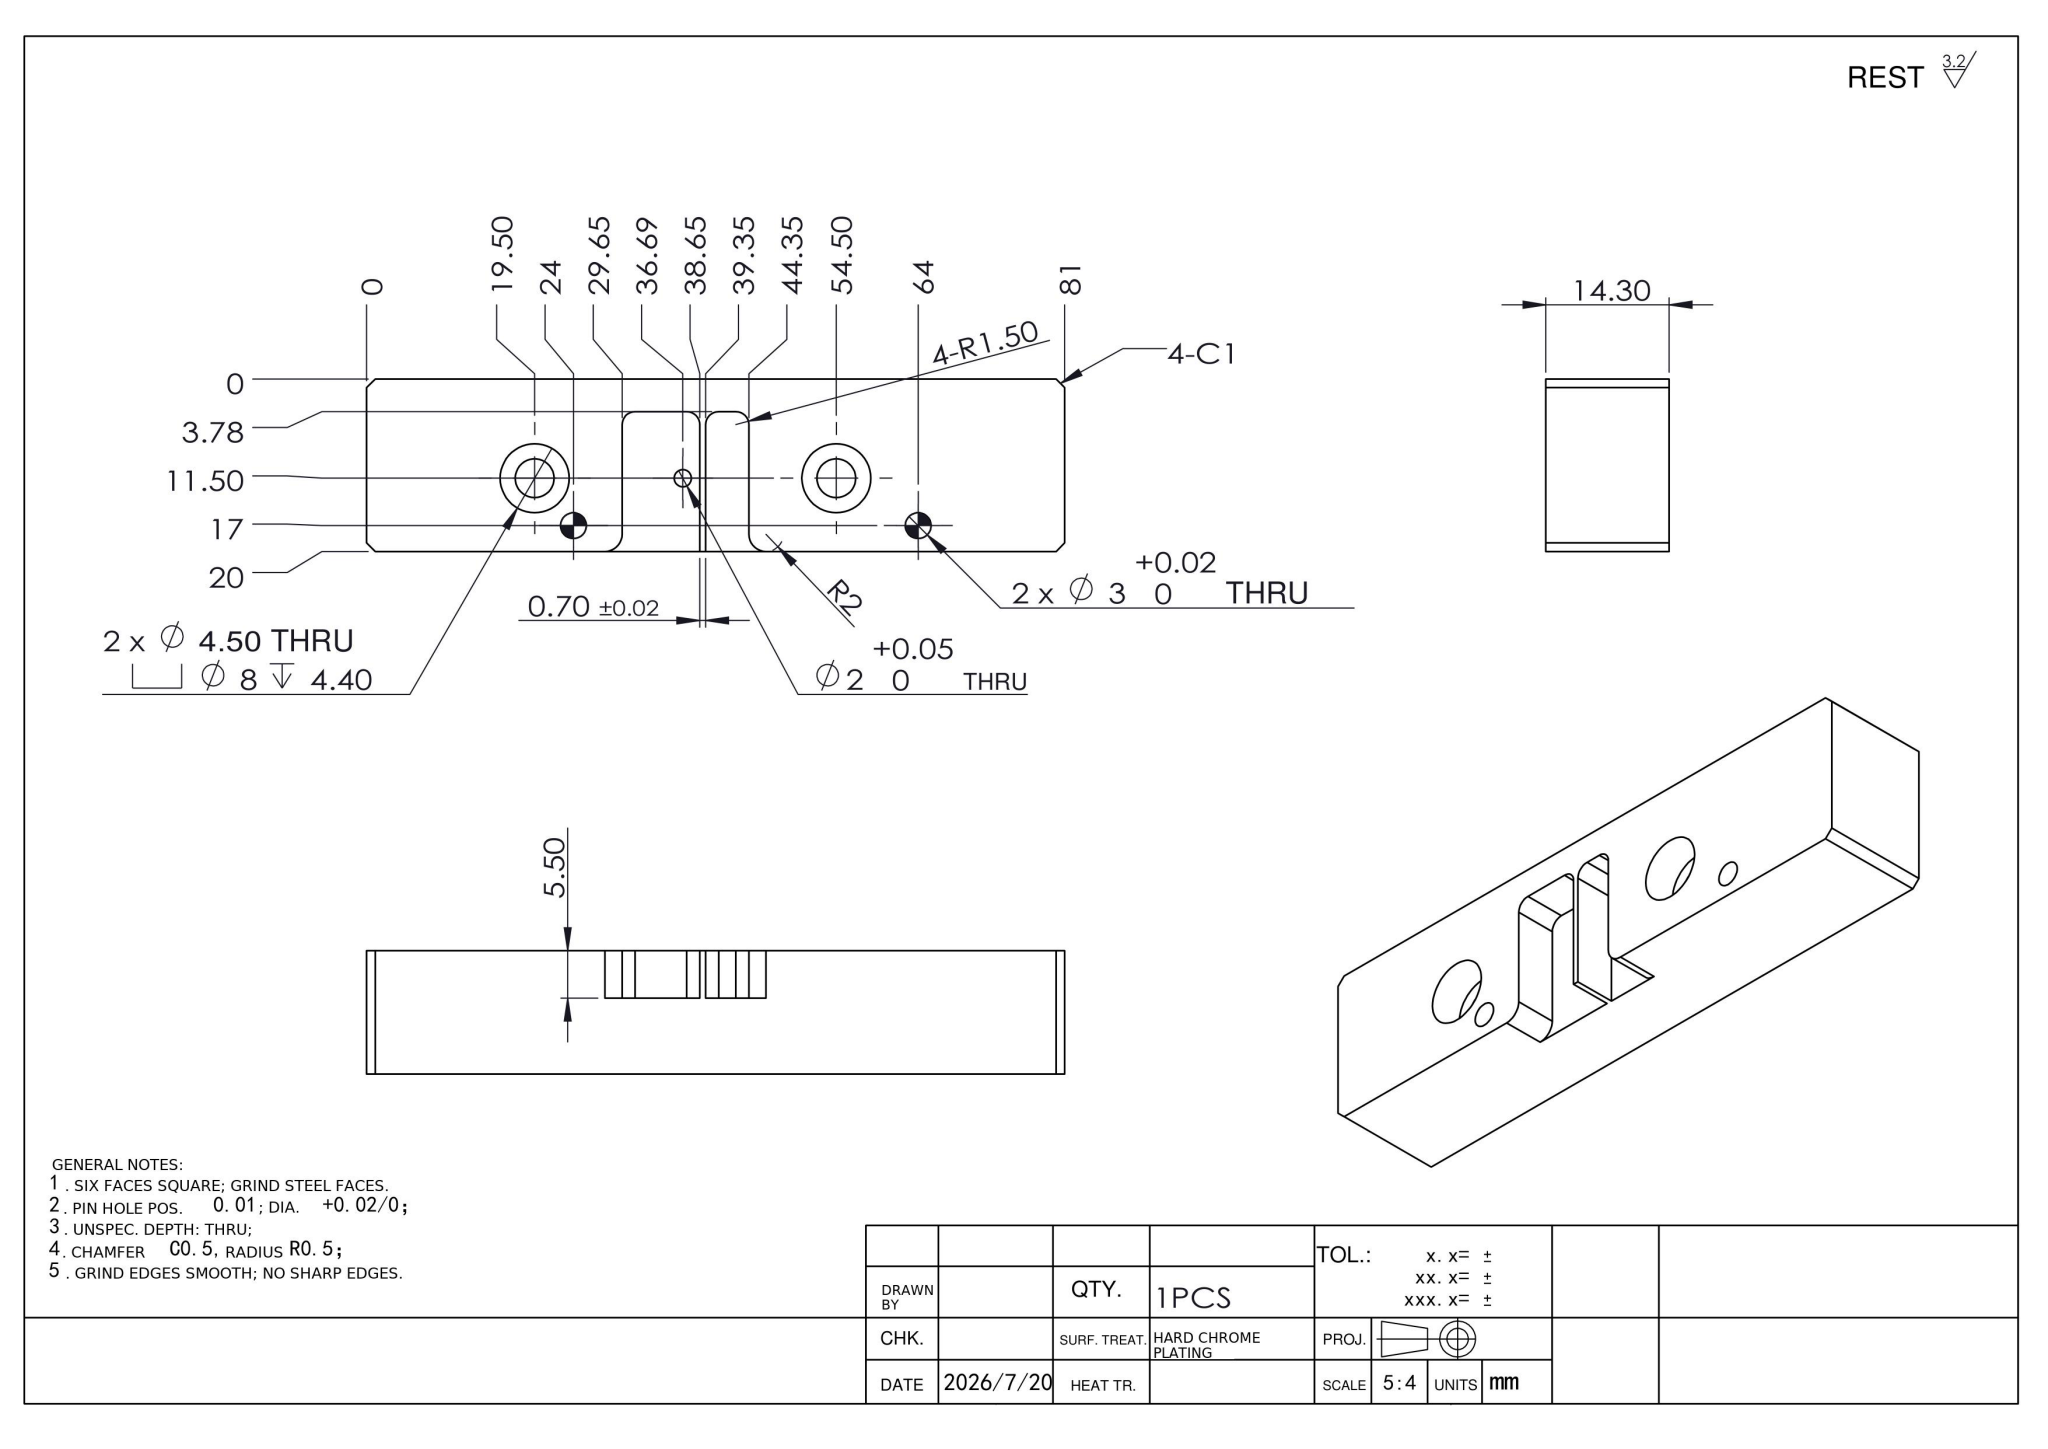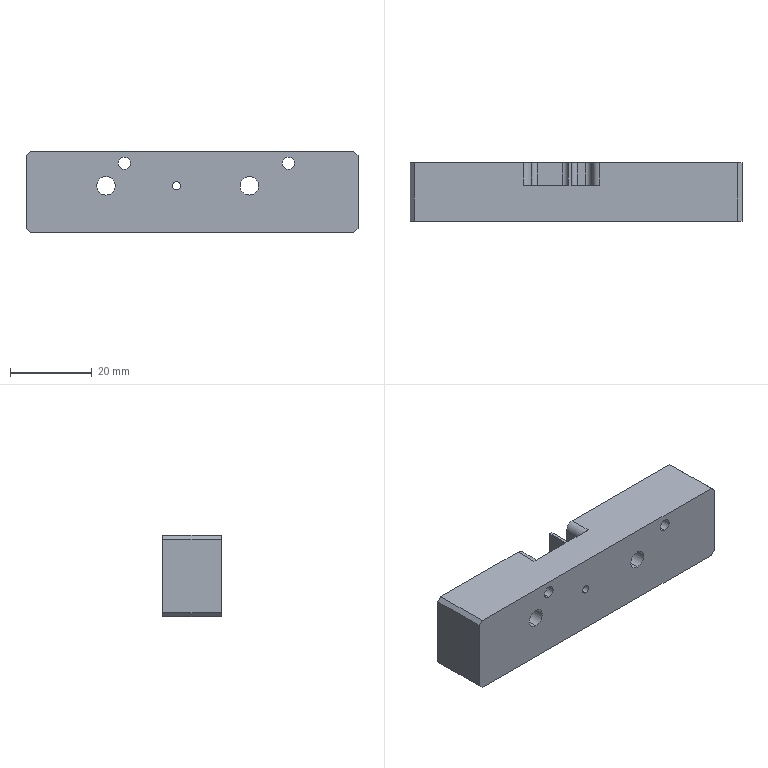Part | NX | mm | 1 solid | 40 faces | box 81 x 14.3 x 20 mm | volume 20903 mm3 | cylinder 20 | plane 20 | commonest cylinder face diameters 3 x8 8 x4 4.5 x4 2 x2 4 x2